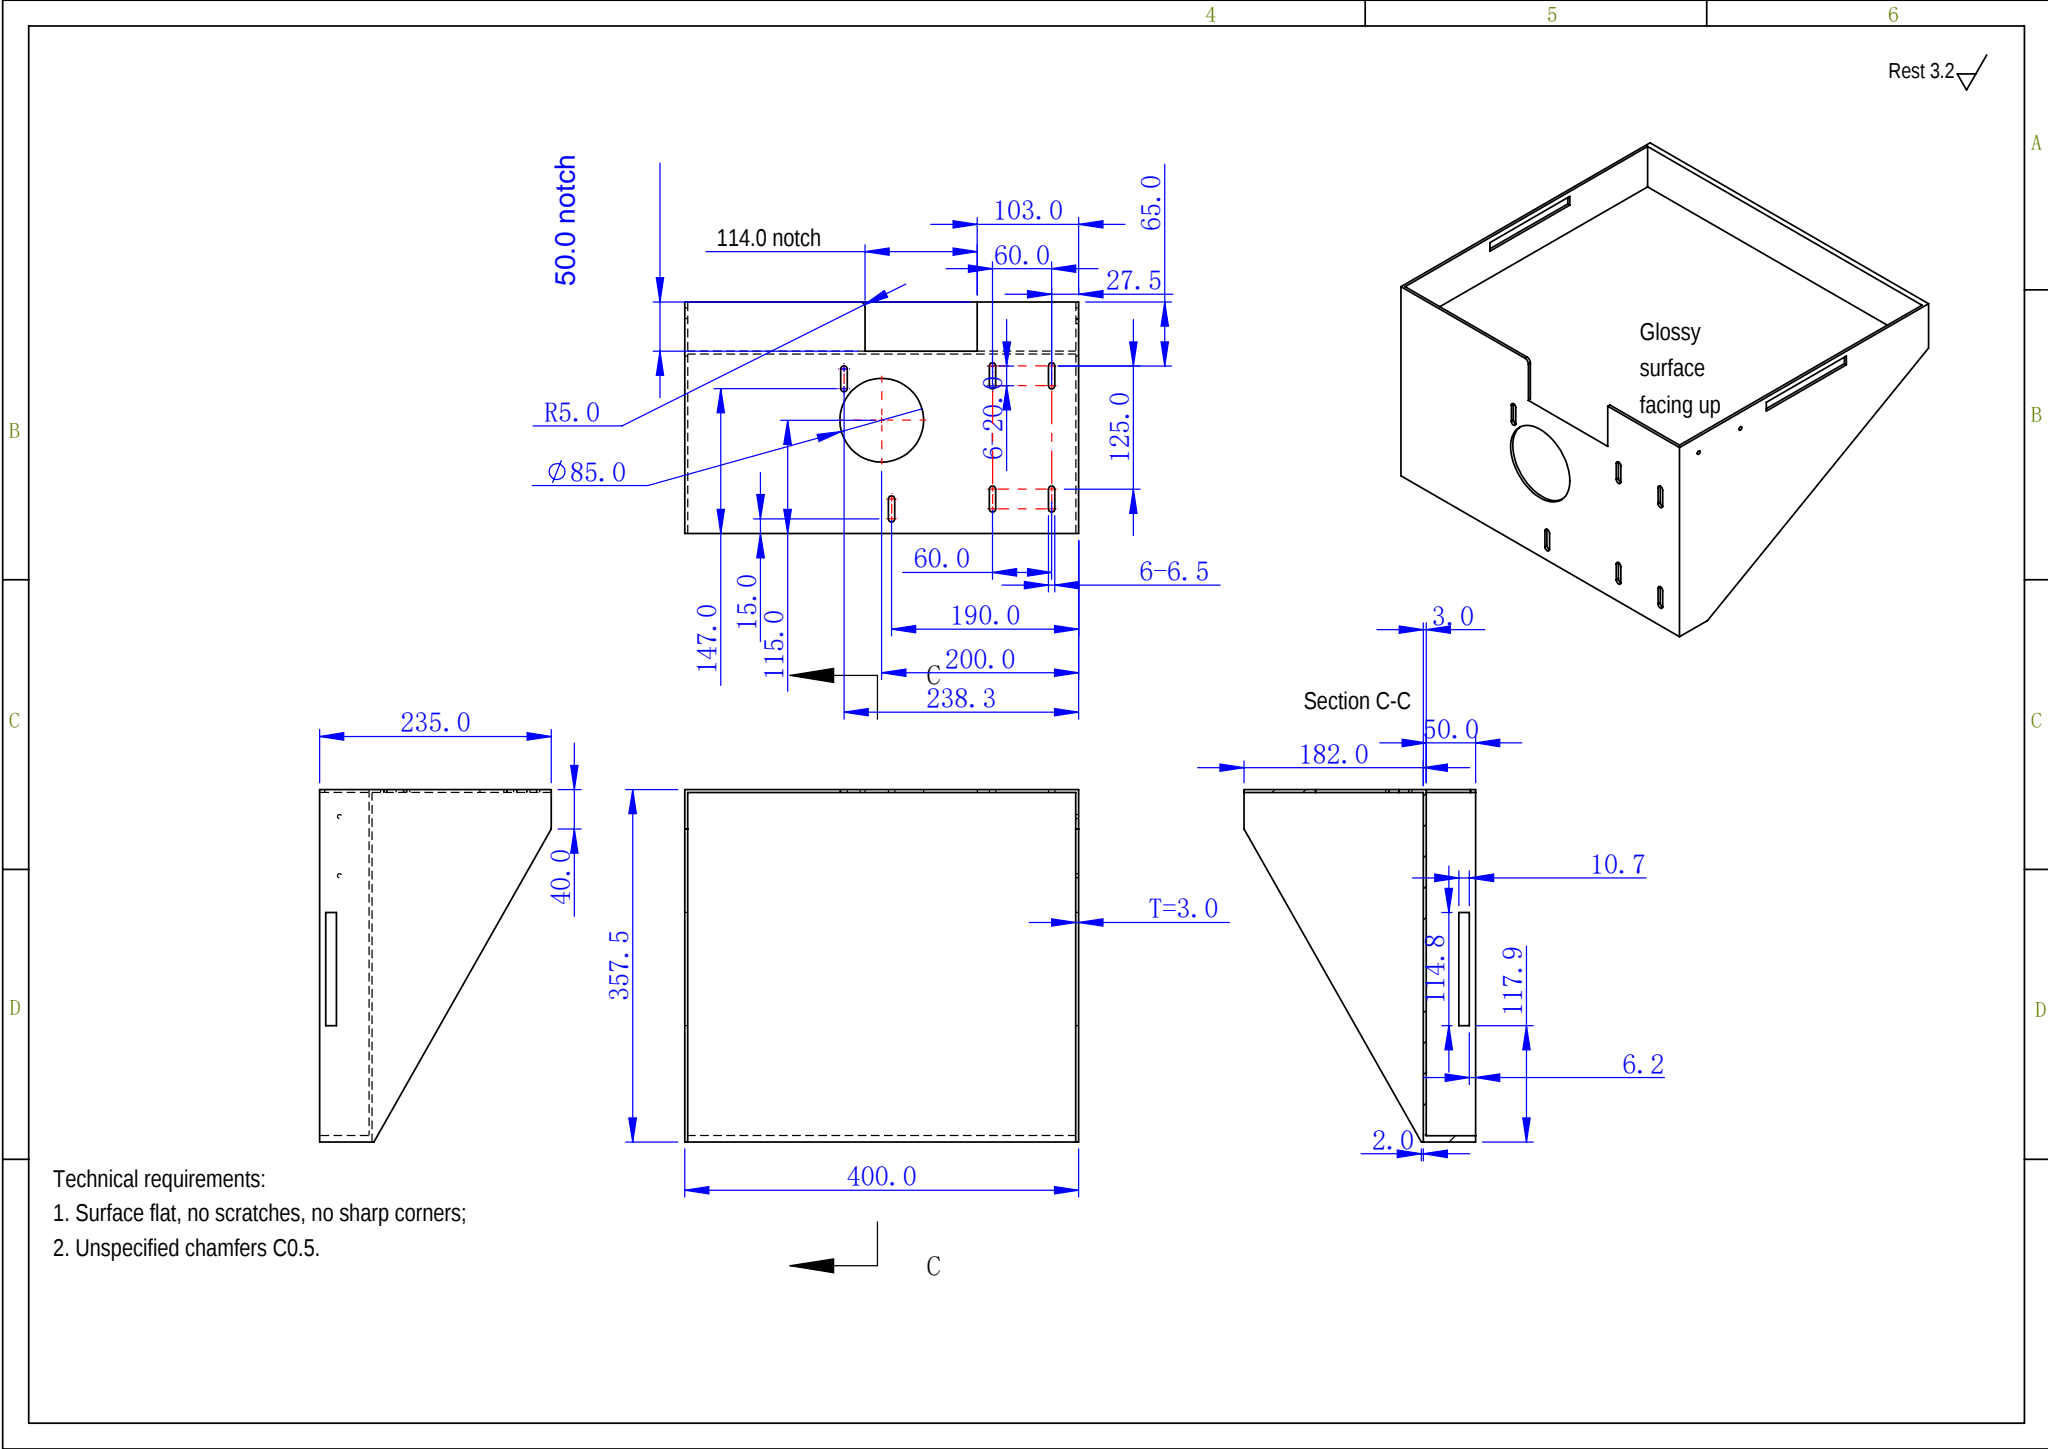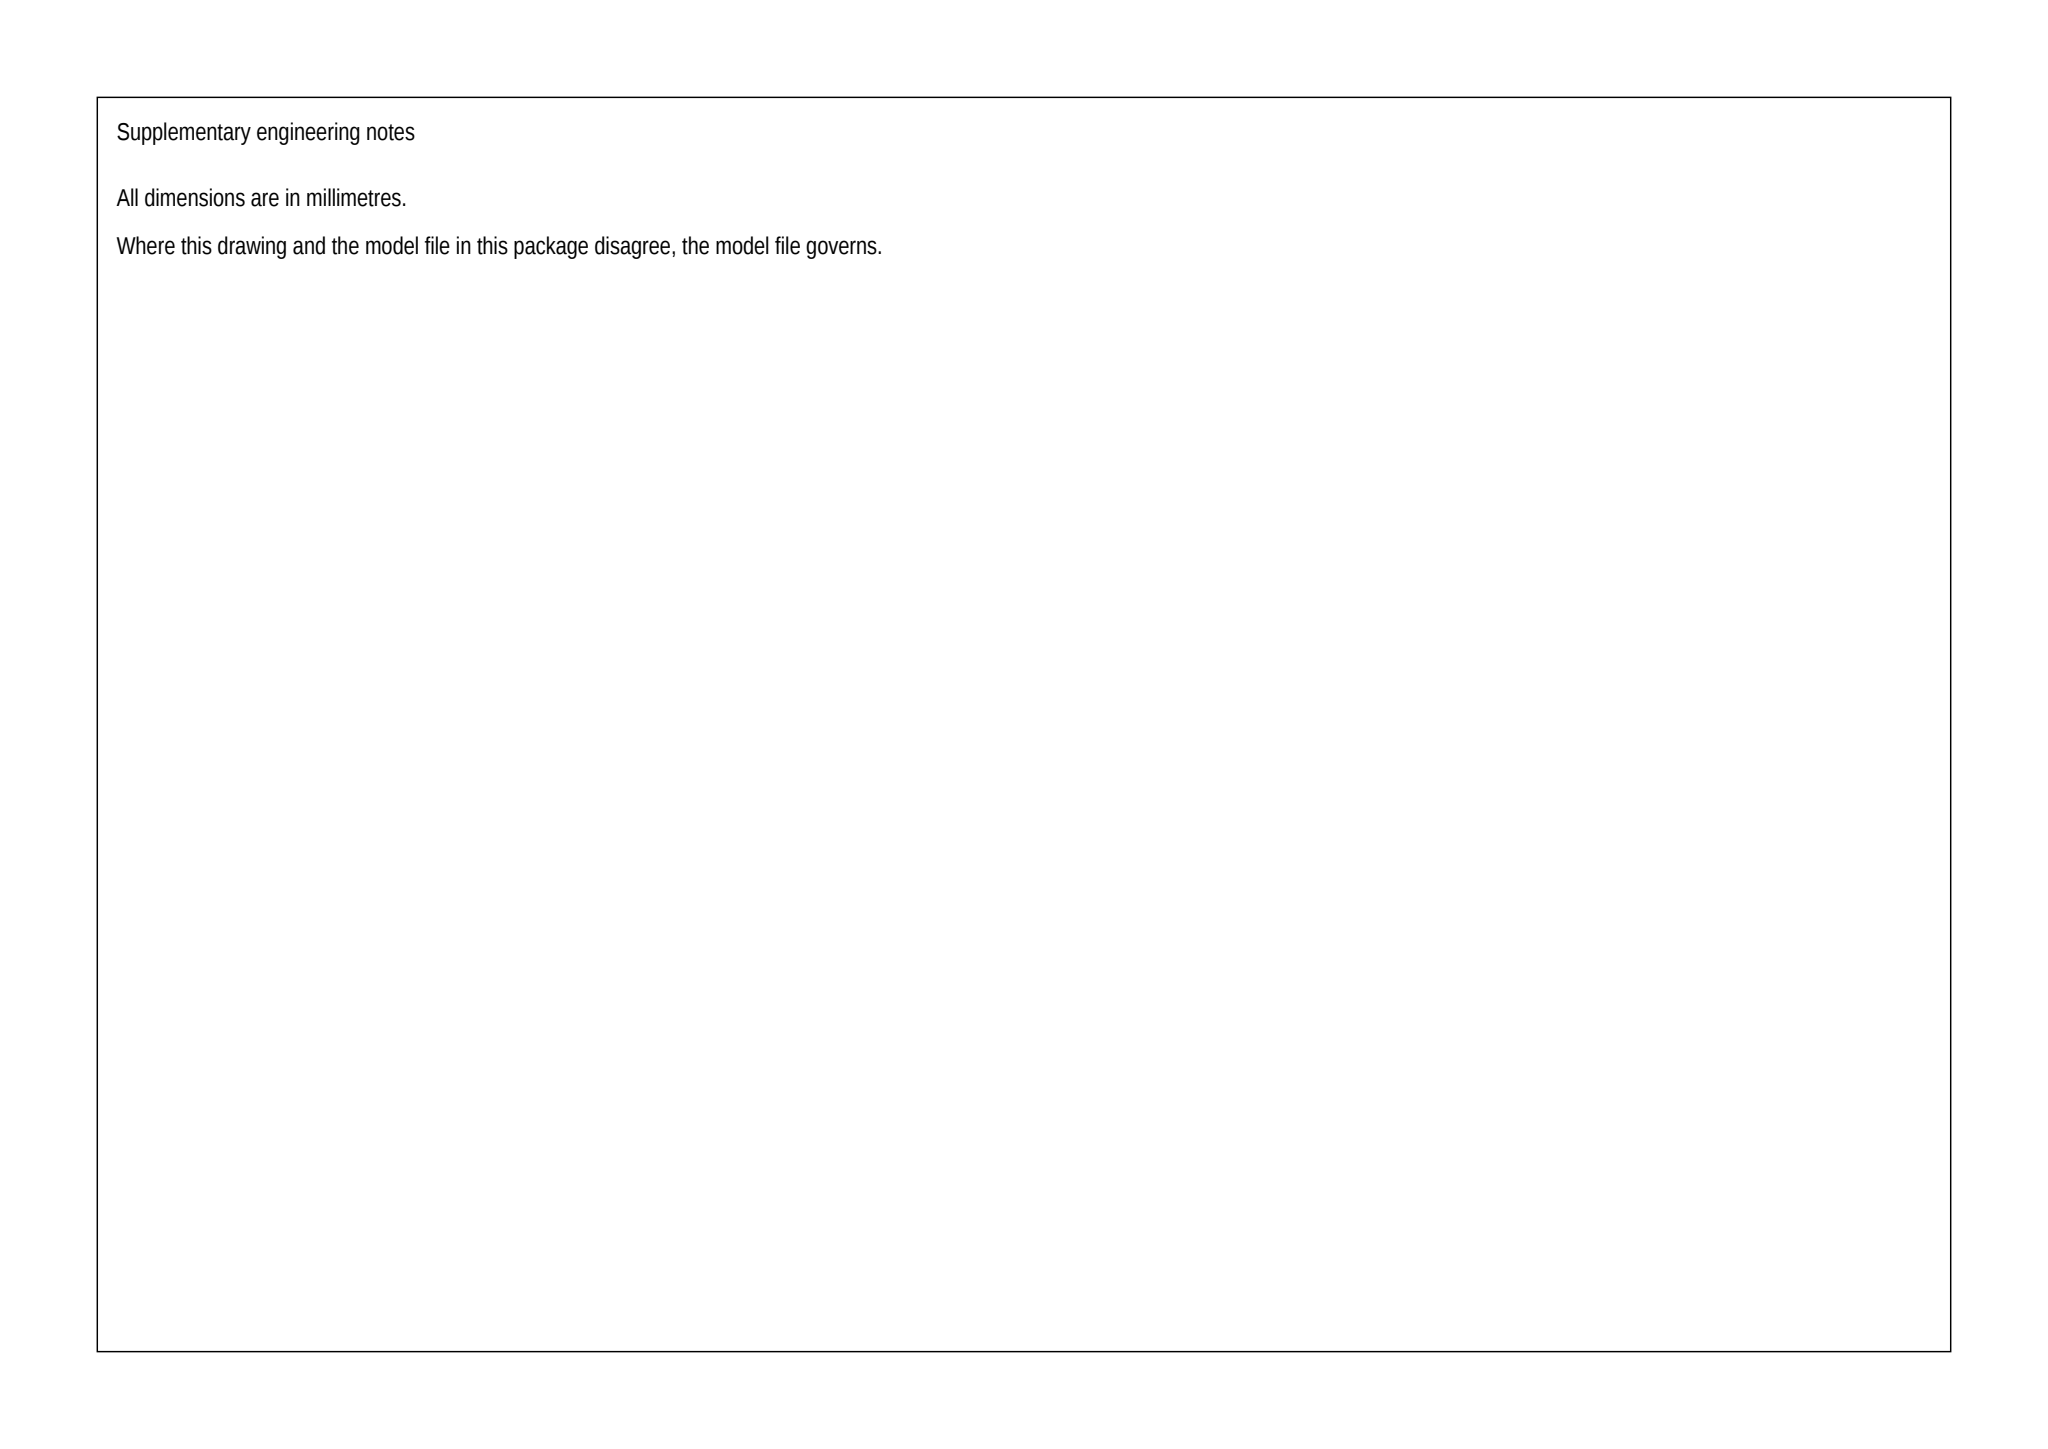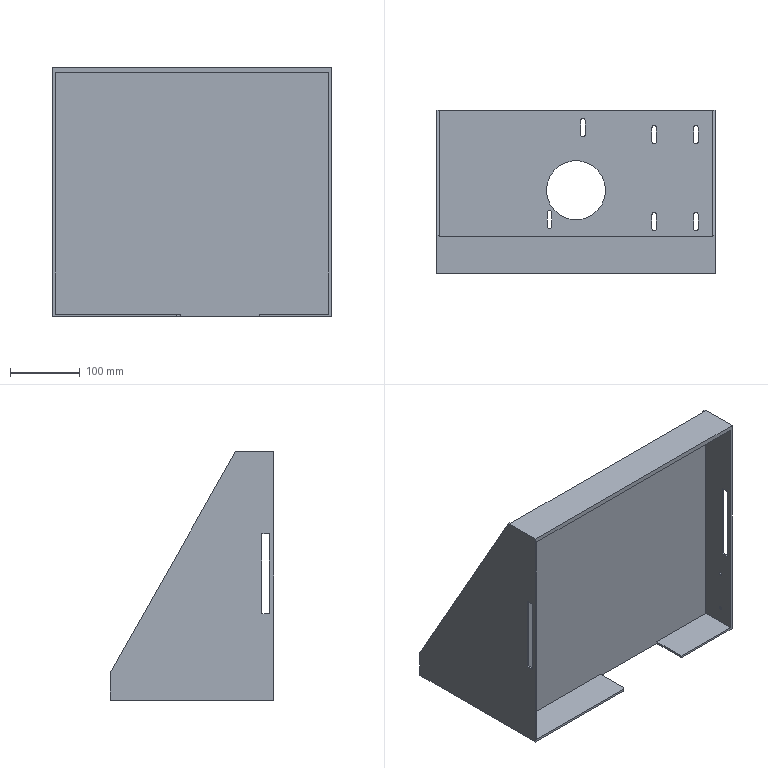Part | SolidWorks | mm | 1 solid | 59 faces | box 400 x 235 x 357.5 mm | volume 1112024 mm3 | plane 40 | cylinder 19 | commonest cylinder face diameters 6.5 x12 4.2 x4 85 x2 10 x1